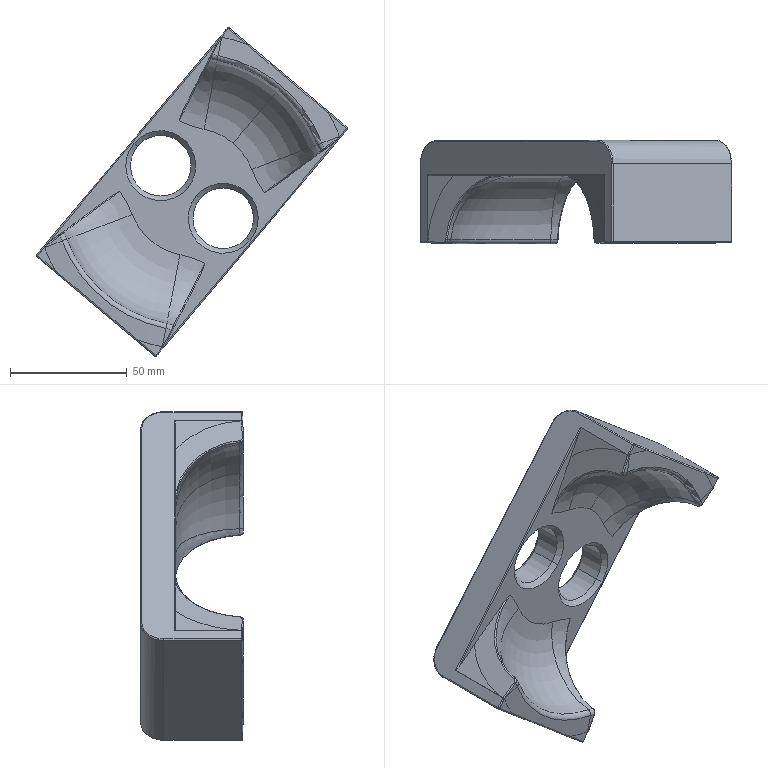Component | SolidWorks | 08ProfileFixture-1 | 1 solid | 120 faces | volume 168391 mm3 | spline 36 | cylinder 31 | cone 22 | torus 13 | plane 11 | sphere 7 | commonest cylinder face diameters 1 x17 6.8 x8 26 x4 20 x2 | material Nylon66